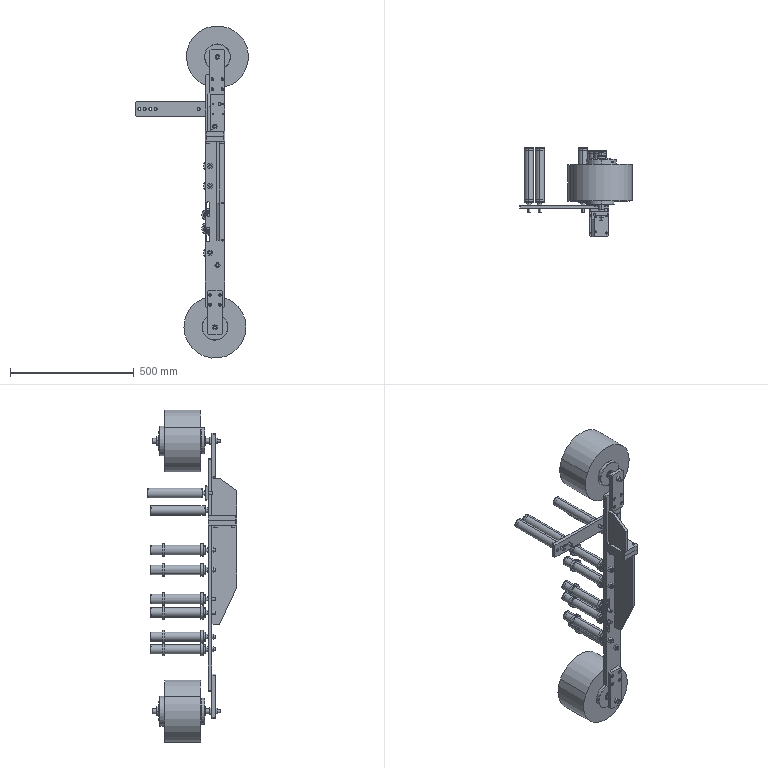Assembly | SolidWorks | mm | 137 component files | 139 solids | 2845 faces | box 455 x 361 x 1340 mm | volume 19278067 mm3 | cylinder 1536 | plane 969 | cone 300 | torus 40 | commonest cylinder face diameters 32 x120 15 x104 33.7 x100 6 x96 28 x80 19 x80 2.5 x80 12 x70
Bill of materials:
8TC-A15004-40-23A | 2 | A3 | Thick annular ring (short hollow cylinder) with small chamfers on its outer edges and one small radial hole through the wall.
8TC-A15004-40-25A | 2 | A3 | Thin flat annular disc (washer-like) with a large central through hole and square-cut edges.
8TC-A15004-80-01A | 1 | A3 | Long, narrow, thin rectangular bar with many through holes of several sizes, two elongated slots, and two blind holes drilled into one narrow end face.
8TC-A15004-80-02A | 2 | A3 | Thick rectangular block plate with two chamfered corners at one end and eight vertical through holes in two sizes.
8TC-A15004-80-03A | 1 | A3 | Flat rectangular bar with one end cut at an angle into a tapered tip, plus two blind holes drilled into the opposite narrow end face.
8TC-A15004-80-04A | 1 | A3 | Flat plate with a five-sided (pentagonal) outline formed by one large angled corner cut. No holes are visible.
8TC-A15004-80-05A | 1 | A3 | Rectangular plate with two chamfered corners at one end and about 13 through holes in roughly three sizes, laid out in a pattern.
8TC-A15004-80-15A | 2 | A3 | Rectangular plate with all four corners chamfered, one larger through hole near one end, and four smaller through holes in a rectangular pattern near the other end.
8TC-A15004-80-16A | 2 | #45 | Stepped cylindrical pin: a long main shaft, a short larger-diameter collar, and a short smaller-diameter stub at one end. The collar appears to have two parallel flats.
8TC-A15004-80-17A | 2 | Black POM | Flanged cylindrical sleeve: a plain cylinder with a thin, larger-diameter flange at one end and a small axial through hole.
8TC-A15004-80-18A | 2 | Black POM | Split ring: an annulus with a single radial slit through the wall and a transverse hole crossing the split region perpendicular to the slit.
8TC-A15004-80-19A | 12 | Black Bakelite | Thin-walled annular ring with small edge chamfers and small radial hole(s) through the wall.
6002 | 20 |  | Short annular ring: a cylinder with a large central through bore and a thin concentric circular line on the end face between the bore and the outer edge.
8TC-A15004-80-13A | 10 | #45 | Long, straight, thin-walled cylindrical tube that is open along its full length.
8TC-A15004-80-14A | 10 | #45 | Long, slender, stepped round shaft. One end has a short small-diameter pin, then a short larger-diameter collar, then a long main shaft that ends in a short reduced or chamfered section.
circlips for hole--type b gb | 20 |  | Thin, flat, open split ring (C-shape) with a circular outer edge and a gap on one side. At each end of the gap the band widens inward into a lug with a small round through-hole. Shape resembles an internal-style retaining ring.
circlips for shaft--type a large gb | 10 |  | Thin, flat, open split ring (C-shape) with a circular inner edge and a narrow straight-sided gap on one side. At each end of the gap the band widens outward into a lug with a small round through-hole. Shape resembles an external-style retaining ring.
M12Nut | 7 | #45 | Hexagonal prism with a plain round through bore on its central axis.
M6x20SocketHeadCapScrew | 23 | #45 | Headed cylindrical pin: a short, larger-diameter cylindrical head joined to a longer, smaller-diameter cylindrical shank with a chamfered free end.
M8x30HexSocketHeadCapScrew | 4 | #45 | Headed cylindrical pin, similar to the previous part: a cylindrical head and a longer, smaller cylindrical shank with a chamfered end. The head is slightly smaller relative to the shank.
Part41 | 1 |  | Flat rectangular bar with small corner chamfers. It has a row of four round through holes near one end, one isolated round hole further along, and four lengthwise slots arranged in a 2x2 pattern near the other end.
ProtectiveFilm | 1 |  | Thick-walled cylindrical bushing or spacer shape: a solid cylinder with a small central through bore.
Mates:
1. coincident | 8TC-A15004-80-01A-1 face at (80, 7.5, 0) dir (0, 0, 1) | 8TC-A15004-80-02A-1 face at (40, -50, 0) dir (0, 0, -1)
2. width | 8TC-A15004-80-01A-1 face at (80, 7.5, -670) dir (1, 0, 0) | 8TC-A15004-80-01A-1 face at (0, 7.5, 0) dir (-1, 0, 0) | 8TC-A15004-80-02A-1 face at (80, -107.5, 0) dir (1, 0, 0) | 8TC-A15004-80-02A-1 face at (0, -107.5, 0) dir (-1, 0, 0)
3. coincident | 8TC-A15004-80-02A-1 face at (40, -50, 0) dir (0, 0, -1) | 8TC-A15004-80-03A-1 face at (60, -107.5, 0) dir (0, 0, 1)
4. coincident | 8TC-A15004-80-01A-1 face at (0, -7.5, 0) dir (0, -1, 0) | 8TC-A15004-80-03A-1 face at (60, -7.5, 0) dir (0, 1, 0)
5. coincident | 8TC-A15004-80-02A-1 face at (0, 7.5, 0) dir (0, 1, 0) | 8TC-A15004-80-02A-2 face at (80, 7.5, 40) dir (0, 1, 0)
6. coincident | 8TC-A15004-80-02A-2 face at (40, -50, 40) dir (0, 0, 1) | 8TC-A15004-80-05A-1 face at (80, -7.5, 40) dir (0, 0, -1)
7. coincident | 8TC-A15004-80-02A-2 face at (80, 7.5, 40) dir (0, 1, 0) | 8TC-A15004-80-05A-1 face at (0, 7.5, 40) dir (0, 1, 0)
8. coincident | 8TC-A15004-80-02A-2 face at (0, -107.5, 40) dir (-1, 0, 0) | 8TC-A15004-80-05A-1 face at (0, -7.5, 40) dir (-1, 0, 0)
9. distance | ProtectiveFilm-1 face at (40, 37.5, -750) dir (0, -1, 0) | 8TC-A15004-80-01A-1 face at (0, 7.5, 0) dir (0, 1, 0)
10. coincident | ProtectiveFilm-1 face at (40, 183.5, -750) dir (0, 1, 0) | ProtectiveFilm-4 face at (50, 183.5, 340) dir (0, 1, 0)
11. concentric | 8TC-A15004-80-01A-1 face at (50, -7.5, -500) dir (0, 1, 0) r 6 | 8TC-A15004-83-00-8/8TC-A15004-80-14A-1 face at (50, -22.5, -500) dir (0, -1, 0) r 6
12. coincident | 8TC-A15004-80-01A-1 face at (0, 7.5, 0) dir (0, 1, 0) | 8TC-A15004-83-00-8/8TC-A15004-80-14A-1 face at (50, 7.5, -505) dir (0, -1, 0)
13. concentric | 8TC-A15004-80-01A-1 face at (20, -7.5, -450) dir (0, 1, 0) r 6 | 8TC-A15004-83-00-9/8TC-A15004-80-14A-1 face at (20, -22.5, -450) dir (0, -1, 0) r 6
14. coincident | 8TC-A15004-80-01A-1 face at (0, 7.5, 0) dir (0, 1, 0) | 8TC-A15004-83-00-9/8TC-A15004-80-14A-1 face at (20, 7.5, -455) dir (0, -1, 0)
15. coincident | 8TC-A15004-80-05A-1 face at (0, 7.5, 40) dir (0, 1, 0) | assembly face at (20, 7.5, 185) dir (0, -1, 0)
16. concentric | 8TC-A15004-80-05A-1 face at (20, 7.5, 190) dir (0, -1, 0) r 10 | assembly face at (20, -22.5, 190) dir (0, -1, 0) r 6
17. coincident | 8TC-A15004-80-01A-1 face at (0, 7.5, 0) dir (0, 1, 0) | assembly face at (40, 7.5, -101.842) dir (0, -1, 0)
18. width | 8TC-A15004-80-01A-1 face at (0, 7.5, 0) dir (-1, 0, 0) | 8TC-A15004-80-01A-1 face at (80, 7.5, -670) dir (1, 0, 0) | assembly face at (15, 22.5, -26.842) dir (-1, 0, 0) | assembly face at (65, 22.5, -26.842) dir (1, 0, 0)
19. coincident | 8TC-A15004-80-01A-1 face at (0, 7.5, 0) dir (0, 1, 0) | assembly face at (40, 7.5, -325) dir (0, -1, 0)
20. width | 8TC-A15004-80-01A-1 face at (80, 7.5, -670) dir (1, 0, 0) | 8TC-A15004-80-01A-1 face at (0, 7.5, 0) dir (-1, 0, 0) | assembly face at (0, 22.5, -415) dir (-1, 0, 0) | assembly face at (80, 22.5, -415) dir (1, 0, 0)
21. distance | assembly face at (80, 22.5, -235) dir (0, 0, 1) | 8TC-A15004-80-02A-1 face at (40, -50, 20) dir (0, 0, 1)
22. concentric | 8TC-A15004-80-01A-1 face at (20, -7.5, -100) dir (0, 1, 0) r 6 | 8TC-A15004-83-00-7/8TC-A15004-80-14A-1 face at (20, -22.5, -100) dir (0, -1, 0) r 6
23. concentric | 8TC-A15004-80-01A-1 face at (20, -7.5, -180) dir (0, 1, 0) r 6 | 8TC-A15004-83-00-6/8TC-A15004-80-14A-1 face at (20, -22.5, -180) dir (0, -1, 0) r 6
24. coincident | 8TC-A15004-80-01A-1 face at (0, 7.5, 0) dir (0, 1, 0) | 8TC-A15004-83-00-6/8TC-A15004-80-14A-1 face at (20, 7.5, -185) dir (0, -1, 0)
25. coincident | 8TC-A15004-80-01A-1 face at (0, 7.5, 0) dir (0, 1, 0) | 8TC-A15004-83-00-7/8TC-A15004-80-14A-1 face at (20, 7.5, -105) dir (0, -1, 0)
26. distance | 8TC-A15004-80-03A-1 face at (60, -7.5, 0) dir (1, 0, 0) | 8TC-A15004-80-01A-1 face at (80, 7.5, -670) dir (1, 0, 0)
27. coincident | 8TC-A15004-80-05A-1 face at (0, -7.5, 40) dir (0, -1, 0) | 8TC-A15004-80-04A-1 face at (10, -7.5, 40) dir (0, 1, 0)
28. coincident | 8TC-A15004-80-02A-2 face at (40, -50, 40) dir (0, 0, 1) | 8TC-A15004-80-04A-1 face at (10, -107.5, 40) dir (0, 0, -1)
29. distance | 8TC-A15004-80-04A-1 face at (10, -7.5, 40) dir (-1, 0, 0) | 8TC-A15004-80-02A-2 face at (0, -107.5, 40) dir (-1, 0, 0)
30. concentric | 8TC-A15004-80-02A-2 face at (26, -87.5, 20) dir (0, 0, -1) r 3.3 | M6x20SocketHeadCapScrew-1 face at (26, -87.5, 46.4) dir (0, 0, 1) r 3
31. coincident | 8TC-A15004-80-02A-2 face at (26, -84.2, 26.4) dir (0, 0, -1) | M6x20SocketHeadCapScrew-1 face at (20.75, -87.5, 26.4) dir (0, 0, 1)
32. concentric | 8TC-A15004-80-02A-2 face at (26, -27.5, 20) dir (0, 0, -1) r 3.3 | M6x20SocketHeadCapScrew-2 face at (26, -27.5, 46.4) dir (0, 0, 1) r 3
33. coincident | 8TC-A15004-80-02A-2 face at (26, -24.2, 26.4) dir (0, 0, -1) | M6x20SocketHeadCapScrew-2 face at (20.75, -27.5, 26.4) dir (0, 0, 1)
34. concentric | 8TC-A15004-80-02A-2 face at (20, 0, 20) dir (0, 0, -1) r 3.3 | M6x20SocketHeadCapScrew-3 face at (20, 0, 46.4) dir (0, 0, 1) r 3
35. coincident | M6x20SocketHeadCapScrew-2 face at (26, -27.5, 20.4) dir (0, 0, -1) | M6x20SocketHeadCapScrew-3 face at (20, 0, 20.4) dir (0, 0, -1)
36. concentric | 8TC-A15004-80-02A-2 face at (60, 0, 20) dir (0, 0, -1) r 3.3 | M6x20SocketHeadCapScrew-4 face at (60, 0, 46.4) dir (0, 0, 1) r 3
37. coincident | M6x20SocketHeadCapScrew-3 face at (20, 0, 20.4) dir (0, 0, -1) | M6x20SocketHeadCapScrew-4 face at (60, 0, 20.4) dir (0, 0, -1)
38. coincident | 8TC-A15004-80-05A-1 face at (19.3, 1.1, 70) dir (0, 1, 0) | M6x20SocketHeadCapScrew-5 face at (10.75, 1.1, 70) dir (0, -1, 0)
39. concentric | 8TC-A15004-80-05A-1 face at (16, 7.5, 70) dir (0, 1, 0) r 3.3 | M6x20SocketHeadCapScrew-5 face at (16, -18.9, 70) dir (0, -1, 0) r 3
40. coincident | M6x20SocketHeadCapScrew-5 face at (16, 7.1, 70) dir (0, 1, 0) | M6x20SocketHeadCapScrew-6 face at (16, 7.1, 120) dir (0, 1, 0)
41. concentric | 8TC-A15004-80-05A-1 face at (16, 7.5, 120) dir (0, 1, 0) r 3.3 | M6x20SocketHeadCapScrew-6 face at (16, -18.9, 120) dir (0, -1, 0) r 3
42. coincident | M6x20SocketHeadCapScrew-6 face at (16, 7.1, 120) dir (0, 1, 0) | M6x20SocketHeadCapScrew-7 face at (16, 7.1, 170) dir (0, 1, 0)
43. concentric | 8TC-A15004-80-05A-1 face at (16, 7.5, 170) dir (0, 1, 0) r 3.3 | M6x20SocketHeadCapScrew-7 face at (16, -18.9, 170) dir (0, -1, 0) r 3
44. coincident | 8TC-A15004-80-05A-1 face at (0, -7.5, 40) dir (0, -1, 0) | M12Nut-1 face at (40, -7.5, 60) dir (0, 1, 0)
45. coincident | 8TC-A15004-80-01A-1 face at (0, -7.5, 0) dir (0, -1, 0) | M12Nut-2 face at (20, -7.5, -100) dir (0, 1, 0)
46. concentric | 8TC-A15004-83-00-7/8TC-A15004-80-14A-1 face at (20, -22.5, -100) dir (0, -1, 0) r 6 | M12Nut-2 face at (20, -7.5, -100) dir (0, 1, 0) r 6
47. coincident | 8TC-A15004-80-01A-1 face at (0, -7.5, 0) dir (0, -1, 0) | M12Nut-13 face at (20, -7.5, -180) dir (0, 1, 0)
48. concentric | 8TC-A15004-83-00-6/8TC-A15004-80-14A-1 face at (20, -22.5, -180) dir (0, -1, 0) r 6 | M12Nut-13 face at (20, -7.5, -180) dir (0, 1, 0) r 6
49. concentric | 8TC-A15004-83-00-9/8TC-A15004-80-14A-1 face at (20, -22.5, -450) dir (0, -1, 0) r 6 | M12Nut-15 face at (20, -7.5, -450) dir (0, 1, 0) r 6
50. coincident | 8TC-A15004-80-01A-1 face at (0, -7.5, 0) dir (0, -1, 0) | M12Nut-15 face at (20, -7.5, -450) dir (0, 1, 0)
51. coincident | 8TC-A15004-80-01A-1 face at (0, -7.5, 0) dir (0, -1, 0) | M12Nut-17 face at (50, -7.5, -500) dir (0, 1, 0)
52. concentric | 8TC-A15004-83-00-8/8TC-A15004-80-14A-1 face at (50, -22.5, -500) dir (0, -1, 0) r 6 | M12Nut-17 face at (50, -7.5, -500) dir (0, 1, 0) r 6
53. coincident | 8TC-A15004-80-02A-1 face at (40, -50, 0) dir (0, 0, -1) | M8x30HexSocketHeadCapScrew-5 face at (3, -92.5, 0) dir (0, 0, 1)
54. concentric | 8TC-A15004-80-02A-1 face at (10, -92.5, 0) dir (0, 0, -1) r 4.5 | M8x30HexSocketHeadCapScrew-5 face at (10, -92.5, 30) dir (0, 0, 1) r 4
55. coincident | 8TC-A15004-80-02A-1 face at (40, -50, 0) dir (0, 0, -1) | M8x30HexSocketHeadCapScrew-13 face at (63, -92.5, 0) dir (0, 0, 1)
56. concentric | 8TC-A15004-80-02A-1 face at (70, -92.5, 0) dir (0, 0, -1) r 4.5 | M8x30HexSocketHeadCapScrew-13 face at (70, -92.5, 30) dir (0, 0, 1) r 4
57. coincident | 8TC-A15004-80-02A-1 face at (40, -50, 0) dir (0, 0, -1) | M8x30HexSocketHeadCapScrew-15 face at (3, -22.5, 0) dir (0, 0, 1)
58. concentric | 8TC-A15004-80-02A-1 face at (10, -22.5, 0) dir (0, 0, -1) r 4.5 | M8x30HexSocketHeadCapScrew-15 face at (10, -22.5, 30) dir (0, 0, 1) r 4
59. concentric | 8TC-A15004-80-02A-1 face at (70, -22.5, 0) dir (0, 0, -1) r 4.5 | M8x30HexSocketHeadCapScrew-17 face at (70, -22.5, 30) dir (0, 0, 1) r 4
60. coincident | 8TC-A15004-80-02A-1 face at (40, -50, 0) dir (0, 0, -1) | M8x30HexSocketHeadCapScrew-17 face at (63, -22.5, 0) dir (0, 0, 1)
61. coincident | 8TC-A15004-80-02A-1 face at (54, -84.2, 13.6) dir (0, 0, 1) | M6x20SocketHeadCapScrew-8 face at (58.85, -85.489, 13.6) dir (0, 0, -1)
62. concentric | 8TC-A15004-80-02A-1 face at (54, -87.5, 20) dir (0, 0, 1) r 3.3 | M6x20SocketHeadCapScrew-8 face at (54, -87.5, -6.4) dir (0, 0, -1) r 3
63. coincident | M6x20SocketHeadCapScrew-8 face at (54, -87.5, 19.6) dir (0, 0, 1) | M6x20SocketHeadCapScrew-40 face at (54, -27.5, 19.6) dir (0, 0, 1)
64. concentric | 8TC-A15004-80-02A-1 face at (54, -27.5, 20) dir (0, 0, 1) r 3.3 | M6x20SocketHeadCapScrew-40 face at (54, -27.5, -6.4) dir (0, 0, -1) r 3
65. coincident | M6x20SocketHeadCapScrew-40 face at (54, -27.5, 19.6) dir (0, 0, 1) | M6x20SocketHeadCapScrew-42 face at (60, 0, 19.6) dir (0, 0, 1)
66. concentric | 8TC-A15004-80-02A-1 face at (60, 0, 20) dir (0, 0, 1) r 3.3 | M6x20SocketHeadCapScrew-42 face at (60, 0, -6.4) dir (0, 0, -1) r 3
67. coincident | M6x20SocketHeadCapScrew-42 face at (60, 0, 19.6) dir (0, 0, 1) | M6x20SocketHeadCapScrew-44 face at (20, 0, 19.6) dir (0, 0, 1)
68. concentric | 8TC-A15004-80-02A-1 face at (20, 0, 20) dir (0, 0, 1) r 3.3 | M6x20SocketHeadCapScrew-44 face at (20, 0, -6.4) dir (0, 0, -1) r 3
69. coincident | 8TC-A15004-80-01A-1 face at (57.3, 1.1, -50) dir (0, 1, 0) | M6x20SocketHeadCapScrew-46 face at (59.09, 1.1, -51.288) dir (0, -1, 0)
70. concentric | 8TC-A15004-80-01A-1 face at (54, 7.5, -50) dir (0, 1, 0) r 3.3 | M6x20SocketHeadCapScrew-46 face at (54, -18.9, -50) dir (0, -1, 0) r 3
71. coincident | M6x20SocketHeadCapScrew-46 face at (54, 7.1, -50) dir (0, 1, 0) | M6x20SocketHeadCapScrew-48 face at (54, 7.1, -150) dir (0, 1, 0)
72. concentric | 8TC-A15004-80-01A-1 face at (54, 7.5, -150) dir (0, 1, 0) r 3.3 | M6x20SocketHeadCapScrew-48 face at (54, -18.9, -150) dir (0, -1, 0) r 3
73. coincident | M6x20SocketHeadCapScrew-48 face at (54, 7.1, -150) dir (0, 1, 0) | M6x20SocketHeadCapScrew-50 face at (54, 7.1, -250) dir (0, 1, 0)
74. concentric | 8TC-A15004-80-01A-1 face at (54, 7.5, -250) dir (0, 1, 0) r 3.3 | M6x20SocketHeadCapScrew-50 face at (54, -18.9, -250) dir (0, -1, 0) r 3
75. coincident | M6x20SocketHeadCapScrew-50 face at (54, 7.1, -250) dir (0, 1, 0) | M6x20SocketHeadCapScrew-52 face at (54, 7.1, -350) dir (0, 1, 0)
76. concentric | 8TC-A15004-80-01A-1 face at (54, 7.5, -350) dir (0, 1, 0) r 3.3 | M6x20SocketHeadCapScrew-52 face at (54, -18.9, -350) dir (0, -1, 0) r 3
77. coincident | assembly face at (40, 236.5, -320) dir (0, 1, 0) | assembly face at (22.25, 236.5, -385) dir (0, -1, 0)
78. concentric | assembly face at (27.5, 236.5, -385) dir (0, 1, 0) r 3.3 | assembly face at (27.5, 216.5, -385) dir (0, -1, 0) r 3
79. concentric | assembly face at (52.5, 236.5, -385) dir (0, 1, 0) r 3.3 | assembly face at (52.5, 216.5, -385) dir (0, -1, 0) r 3
80. coincident | assembly face at (40, 236.5, -320) dir (0, 1, 0) | assembly face at (47.25, 236.5, -385) dir (0, -1, 0)
81. concentric | assembly face at (27.5, 236.5, -255) dir (0, 1, 0) r 3.3 | assembly face at (27.5, 216.5, -255) dir (0, -1, 0) r 3
82. coincident | assembly face at (40, 236.5, -320) dir (0, 1, 0) | assembly face at (22.25, 236.5, -255) dir (0, -1, 0)
83. coincident | assembly face at (40, 236.5, -320) dir (0, 1, 0) | assembly face at (47.25, 236.5, -255) dir (0, -1, 0)
84. concentric | assembly face at (52.5, 236.5, -255) dir (0, 1, 0) r 3.3 | assembly face at (52.5, 216.5, -255) dir (0, -1, 0) r 3
85. coincident | assembly face at (49.2, 31.1, -320) dir (0, 1, 0) | assembly face at (47.25, 31.1, -320) dir (0, -1, 0)
86. concentric | assembly face at (52.5, 37.5, -320) dir (0, 1, 0) r 3.3 | assembly face at (52.5, 11.1, -320) dir (0, -1, 0) r 3
87. coincident | assembly face at (52.5, 37.1, -320) dir (0, 1, 0) | assembly face at (87.633, 37.1, -298.125) dir (0, 1, 0)
88. coincident | assembly face at (52.5, 37.1, -320) dir (0, 1, 0) | assembly face at (27.5, 37.1, -320) dir (0, 1, 0)
89. coincident | assembly face at (52.5, 37.1, -320) dir (0, 1, 0) | assembly face at (52.5, 37.1, -220) dir (0, 1, 0)
90. coincident | assembly face at (52.5, 37.1, -320) dir (0, 1, 0) | assembly face at (27.5, 37.1, -220) dir (0, 1, 0)
91. concentric | assembly face at (27.5, 11.1, -320) dir (0, -1, 0) r 3 | assembly face at (27.5, 37.5, -320) dir (0, 1, 0) r 3.3
92. concentric | assembly face at (52.5, 11.1, -220) dir (0, -1, 0) r 3 | assembly face at (52.5, 37.5, -220) dir (0, 1, 0) r 3.3
93. concentric | assembly face at (27.5, 37.5, -220) dir (0, 1, 0) r 3.3 | assembly face at (27.5, 11.1, -220) dir (0, -1, 0) r 3
94. concentric | ProtectiveFilm-1 face at (40, 183.5, -750) dir (0, -1, 0) r 38.5 | assembly face at (150, -7.5, -640) dir (0, -1, 0) r 7.5
95. coincident | 8TC-A15004-80-15A-4 face at (30, -16.1, 213.3) dir (0, -1, 0) | M6x20SocketHeadCapScrew-54 face at (25.605, -16.1, 207.129) dir (0, 1, 0)
96. concentric | 8TC-A15004-80-15A-4 face at (30, -22.5, 210) dir (0, -1, 0) r 3.3 | M6x20SocketHeadCapScrew-54 face at (30, 3.9, 210) dir (0, 1, 0) r 3
97. coincident | M6x20SocketHeadCapScrew-54 face at (30, -22.1, 210) dir (0, -1, 0) | M6x20SocketHeadCapScrew-55 face at (70, -22.1, 250) dir (0, -1, 0)
98. coincident | M6x20SocketHeadCapScrew-55 face at (70, -22.1, 250) dir (0, -1, 0) | M6x20SocketHeadCapScrew-56 face at (70, -22.1, 210) dir (0, -1, 0)
99. coincident | M6x20SocketHeadCapScrew-55 face at (70, -22.1, 250) dir (0, -1, 0) | M6x20SocketHeadCapScrew-57 face at (30, -22.1, 250) dir (0, -1, 0)
100. concentric | 8TC-A15004-80-15A-4 face at (30, -22.5, 250) dir (0, -1, 0) r 3.3 | M6x20SocketHeadCapScrew-57 face at (30, 3.9, 250) dir (0, 1, 0) r 3
101. coincident | 8TC-A15004-80-15A-5 face at (20, -16.1, -623.3) dir (0, -1, 0) | M6x20SocketHeadCapScrew-58 face at (15.605, -16.1, -662.871) dir (0, 1, 0)
102. coincident | 8TC-A15004-80-15A-5 face at (60, -16.1, -623.3) dir (0, -1, 0) | M6x20SocketHeadCapScrew-60 face at (15.605, -16.1, -622.871) dir (0, 1, 0)
103. coincident | 8TC-A15004-80-15A-5 face at (60, -16.1, -663.3) dir (0, -1, 0) | M6x20SocketHeadCapScrew-62 face at (55.605, -16.1, -622.871) dir (0, 1, 0)
104. coincident | 8TC-A15004-80-15A-5 face at (20, -16.1, -663.3) dir (0, -1, 0) | M6x20SocketHeadCapScrew-64 face at (55.605, -16.1, -662.871) dir (0, 1, 0)
105. concentric | 8TC-A15004-80-15A-4 face at (50, -7.5, 340) dir (0, -1, 0) r 6 | 8TC-A15004-80-16A-4 face at (50, -42.5, 340) dir (0, -1, 0) r 6
106. coincident | 8TC-A15004-80-01A-1 face at (0, -7.5, 0) dir (0, -1, 0) | 8TC-A15004-80-15A-5 face at (40, -7.5, -690) dir (0, 1, 0)
107. coincident | 8TC-A15004-80-15A-5 face at (40, -22.5, -690) dir (0, -1, 0) | M12Nut-19 face at (40, -22.5, -750) dir (0, 1, 0)
108. concentric | 8TC-A15004-80-15A-5 face at (40, -7.5, -750) dir (0, -1, 0) r 6 | M12Nut-19 face at (40, -30.5, -750) dir (0, -1, 0) r 6
109. coincident | 8TC-A15004-80-15A-5 face at (40, -7.5, -690) dir (0, 1, 0) | 8TC-A15004-80-16A-3 face at (40.526, -7.5, -745.028) dir (0, -1, 0)
110. concentric | 8TC-A15004-80-16A-3 face at (40, -42.5, -750) dir (0, -1, 0) r 6 | M12Nut-19 face at (40, -30.5, -750) dir (0, -1, 0) r 6
111. coincident | ProtectiveFilm-1 face at (40, 37.5, -750) dir (0, -1, 0) | 8TC-A15004-80-17A-1 face at (40, 37.5, -788.5) dir (0, 1, 0)
112. concentric | ProtectiveFilm-1 face at (40, 183.5, -750) dir (0, -1, 0) r 38.5 | 8TC-A15004-80-17A-1 face at (40, 22.5, -750) dir (0, -1, 0) r 38.5
113. concentric | 8TC-A15004-80-17A-1 face at (40, 22.5, -750) dir (0, -1, 0) r 38.5 | 8TC-A15004-80-18A-1 face at (40, 203.5, -750) dir (0, -1, 0) r 38.5
114. coincident | ProtectiveFilm-1 face at (40, 183.5, -750) dir (0, 1, 0) | 8TC-A15004-80-18A-1 face at (40, 183.5, -750) dir (0, -1, 0)
115. concentric | 8TC-A15004-80-16A-3 face at (40, -42.5, -750) dir (0, -1, 0) r 10 | 8TC-A15004-40-23A-1 face at (40, 207.5, -750) dir (0, 1, 0) r 10
116. coincident | 8TC-A15004-80-17A-1 face at (40, 207.5, -760) dir (0, 1, 0) | 8TC-A15004-40-23A-1 face at (40, 207.5, -750) dir (0, -1, 0)
117. concentric | 8TC-A15004-80-16A-3 face at (40, -42.5, -750) dir (0, -1, 0) r 10 | 8TC-A15004-40-25A-1 face at (40, 22.5, -750) dir (0, -1, 0) r 10.25
118. coincident | 8TC-A15004-80-17A-1 face at (40, 22.5, -802.5) dir (0, -1, 0) | 8TC-A15004-40-25A-1 face at (40, 22.5, -750) dir (0, 1, 0)
119. coincident | 8TC-A15004-80-05A-1 face at (0, -7.5, 40) dir (0, -1, 0) | 8TC-A15004-80-15A-4 face at (50, -7.5, 280) dir (0, 1, 0)
120. coincident | 8TC-A15004-80-15A-4 face at (50, -22.5, 280) dir (0, -1, 0) | M12Nut-21 face at (50, -22.5, 340) dir (0, 1, 0)
121. concentric | 8TC-A15004-80-15A-4 face at (50, -7.5, 340) dir (0, -1, 0) r 6 | M12Nut-21 face at (50, -30.5, 340) dir (0, -1, 0) r 6
122. coincident | 8TC-A15004-80-15A-4 face at (50, -7.5, 280) dir (0, 1, 0) | 8TC-A15004-80-16A-4 face at (50, -7.5, 345) dir (0, -1, 0)
123. concentric | 8TC-A15004-80-16A-4 face at (50, -42.5, 340) dir (0, -1, 0) r 10 | 8TC-A15004-80-17A-2 face at (50, 22.5, 340) dir (0, -1, 0) r 38.5
124. coincident | ProtectiveFilm-4 face at (50, 37.5, 340) dir (0, -1, 0) | 8TC-A15004-80-17A-2 face at (50, 37.5, 301.5) dir (0, 1, 0)
125. concentric | 8TC-A15004-80-17A-2 face at (50, 22.5, 340) dir (0, -1, 0) r 38.5 | 8TC-A15004-80-18A-2 face at (50, 203.5, 340) dir (0, -1, 0) r 38.5
126. coincident | ProtectiveFilm-4 face at (50, 183.5, 340) dir (0, 1, 0) | 8TC-A15004-80-18A-2 face at (50, 183.5, 340) dir (0, -1, 0)
127. concentric | 8TC-A15004-80-16A-4 face at (50, -42.5, 340) dir (0, -1, 0) r 10 | 8TC-A15004-40-23A-2 face at (50, 207.5, 340) dir (0, 1, 0) r 10
128. coincident | 8TC-A15004-80-17A-2 face at (50, 207.5, 330) dir (0, 1, 0) | 8TC-A15004-40-23A-2 face at (50, 207.5, 340) dir (0, -1, 0)
129. coincident | 8TC-A15004-80-17A-2 face at (50, 22.5, 287.5) dir (0, -1, 0) | 8TC-A15004-40-25A-2 face at (50, 22.5, 340) dir (0, 1, 0)
130. concentric | 8TC-A15004-80-16A-4 face at (50, -42.5, 340) dir (0, -1, 0) r 10 | 8TC-A15004-40-25A-2 face at (50, 22.5, 340) dir (0, -1, 0) r 10.25
131. concentric | 8TC-A15004-83-00-8/8TC-A15004-80-13A-1 face at (50, 100.224, -500) dir (0, -1, 0) r 19 | 8TC-A15004-80-19A-1 face at (50, 193.5, -500) dir (0, -1, 0) r 19.05
132. coincident | ProtectiveFilm-1 face at (40, 183.5, -750) dir (0, 1, 0) | 8TC-A15004-80-19A-1 face at (50, 183.5, -500) dir (0, -1, 0)
133. concentric | 8TC-A15004-83-00-8/8TC-A15004-80-13A-1 face at (50, 100.224, -500) dir (0, -1, 0) r 19 | 8TC-A15004-80-19A-2 face at (50, 37.5, -500) dir (0, -1, 0) r 19.05
134. coincident | ProtectiveFilm-1 face at (40, 37.5, -750) dir (0, -1, 0) | 8TC-A15004-80-19A-2 face at (50, 37.5, -500) dir (0, 1, 0)
135. concentric | 8TC-A15004-83-00-9/8TC-A15004-80-13A-1 face at (20, 100.224, -450) dir (0, -1, 0) r 19 | 8TC-A15004-80-19A-3 face at (20, 193.5, -450) dir (0, -1, 0) r 19.05
136. coincident | 8TC-A15004-80-19A-1 face at (50, 183.5, -500) dir (0, -1, 0) | 8TC-A15004-80-19A-3 face at (20, 183.5, -450) dir (0, -1, 0)
137. concentric | 8TC-A15004-83-00-9/8TC-A15004-80-13A-1 face at (20, 100.224, -450) dir (0, -1, 0) r 19 | 8TC-A15004-80-19A-4 face at (20, 37.5, -450) dir (0, -1, 0) r 19.05
138. coincident | 8TC-A15004-80-19A-2 face at (50, 37.5, -500) dir (0, 1, 0) | 8TC-A15004-80-19A-4 face at (20, 37.5, -450) dir (0, 1, 0)
139. concentric | 8TC-A15004-83-00-6/8TC-A15004-80-13A-1 face at (20, 100.224, -180) dir (0, -1, 0) r 19 | 8TC-A15004-80-19A-5 face at (20, 193.5, -180) dir (0, -1, 0) r 19.05
140. coincident | 8TC-A15004-80-19A-3 face at (20, 183.5, -450) dir (0, -1, 0) | 8TC-A15004-80-19A-5 face at (20, 183.5, -180) dir (0, -1, 0)
141. concentric | 8TC-A15004-83-00-6/8TC-A15004-80-13A-1 face at (20, 100.224, -180) dir (0, -1, 0) r 19 | 8TC-A15004-80-19A-6 face at (20, 37.5, -180) dir (0, -1, 0) r 19.05
142. coincident | 8TC-A15004-80-19A-4 face at (20, 37.5, -450) dir (0, 1, 0) | 8TC-A15004-80-19A-6 face at (20, 37.5, -180) dir (0, 1, 0)
143. concentric | 8TC-A15004-83-00-7/8TC-A15004-80-13A-1 face at (20, 100.224, -100) dir (0, -1, 0) r 19 | 8TC-A15004-80-19A-7 face at (20, 193.5, -100) dir (0, -1, 0) r 19.05
144. coincident | 8TC-A15004-80-19A-5 face at (20, 183.5, -180) dir (0, -1, 0) | 8TC-A15004-80-19A-7 face at (20, 183.5, -100) dir (0, -1, 0)
145. concentric | 8TC-A15004-83-00-7/8TC-A15004-80-13A-1 face at (20, 100.224, -100) dir (0, -1, 0) r 19 | 8TC-A15004-80-19A-8 face at (20, 37.5, -100) dir (0, -1, 0) r 19.05
146. coincident | 8TC-A15004-80-19A-6 face at (20, 37.5, -180) dir (0, 1, 0) | 8TC-A15004-80-19A-8 face at (20, 37.5, -100) dir (0, 1, 0)
147. concentric | 8TC-A15004-80-05A-1 face at (40, 7.5, 60) dir (0, 1, 0) r 6 | 8TC-A15004-83-00-16/8TC-A15004-80-14A-1 face at (40, -22.5, 60) dir (0, -1, 0) r 6
148. coincident | 8TC-A15004-80-05A-1 face at (0, 7.5, 40) dir (0, 1, 0) | 8TC-A15004-83-00-16/8TC-A15004-80-14A-1 face at (40, 7.5, 55) dir (0, -1, 0)
149. concentric | 8TC-A15004-80-01A-1 face at (20, 7.5, -620) dir (0, 1, 0) r 3 | 8TC-A15004-80-15A-5 face at (20, -22.5, -620) dir (0, -1, 0) r 3.3
150. concentric | 8TC-A15004-80-01A-1 face at (60, 7.5, -660) dir (0, 1, 0) r 3 | 8TC-A15004-80-15A-5 face at (60, -22.5, -660) dir (0, -1, 0) r 3.3
151. concentric | 8TC-A15004-80-16A-3 face at (40, -42.5, -750) dir (0, -1, 0) r 10 | 8TC-A15004-80-17A-1 face at (40, 22.5, -750) dir (0, -1, 0) r 10
152. distance | assembly face at (-590, 112.5, 90) dir (1, 0, 0) | 8TC-A15004-80-02A-3 face at (-530, -107.5, 0) dir (-1, 0, 0)
153. concentric | ProtectiveFilm-4 face at (50, 183.5, 340) dir (0, -1, 0) r 38.5 | 8TC-A15004-80-17A-2 face at (50, 22.5, 340) dir (0, -1, 0) r 38.5
154. concentric | M12Nut-1 face at (40, -7.5, 60) dir (0, 1, 0) r 6 | 8TC-A15004-83-00-16/8TC-A15004-80-14A-1 face at (40, -22.5, 60) dir (0, -1, 0) r 6
155. concentric | 8TC-A15004-80-05A-1 face at (70, 7.5, 250) dir (0, 1, 0) r 3 | M6x20SocketHeadCapScrew-55 face at (70, 3.9, 250) dir (0, 1, 0) r 3
156. distance | 8TC-A15004-80-05A-1 face at (0, -7.5, 270) dir (0, 0, 1) | 8TC-A15004-80-15A-4 face at (80, -22.5, 190) dir (0, 0, -1)
157. coincident | 8TC-A15004-80-05A-1 face at (80, -7.5, 270) dir (1, 0, 0) | 8TC-A15004-80-15A-4 face at (80, -22.5, 190) dir (1, 0, 0)
158. coincident | 8TC-A15004-80-01A-1 face at (0, 7.5, 0) dir (0, 1, 0) | 8TC-A15004-83-00-17/8TC-A15004-80-14A-1 face at (13, 7.5, -302.5) dir (0, -1, 0)
159. slot | 8TC-A15004-83-00-17/8TC-A15004-80-14A-1 face at (13, -22.5, -297.5) dir (0, -1, 0) r 6 | 8TC-A15004-80-01A-1 face at (19, -7.5, -297.5) dir (-1, 0, 0)
160. coincident | 8TC-A15004-80-01A-1 face at (0, 7.5, 0) dir (0, 1, 0) | 8TC-A15004-83-00-18/8TC-A15004-80-14A-1 face at (13, 7.5, -357.5) dir (0, -1, 0)
161. slot | 8TC-A15004-83-00-18/8TC-A15004-80-14A-1 face at (13, -22.5, -352.5) dir (0, -1, 0) r 6 | 8TC-A15004-80-01A-1 face at (19, -7.5, -352.5) dir (-1, 0, 0)
162. concentric | 8TC-A15004-83-00-18/8TC-A15004-80-13A-1 face at (13, 100.224, -352.5) dir (0, -1, 0) r 19 | 8TC-A15004-80-19A-17 face at (13, 193.5, -352.5) dir (0, -1, 0) r 19.05
163. coincident | 8TC-A15004-80-19A-3 face at (20, 193.5, -450) dir (0, 1, 0) | 8TC-A15004-80-19A-17 face at (13, 193.5, -352.5) dir (0, 1, 0)
164. concentric | 8TC-A15004-83-00-17/8TC-A15004-80-13A-1 face at (13, 100.224, -297.5) dir (0, -1, 0) r 19 | 8TC-A15004-80-19A-18 face at (13, 193.5, -297.5) dir (0, -1, 0) r 19.05
165. coincident | 8TC-A15004-80-19A-17 face at (13, 193.5, -352.5) dir (0, 1, 0) | 8TC-A15004-80-19A-18 face at (13, 193.5, -297.5) dir (0, 1, 0)
166. concentric | 8TC-A15004-83-00-17/8TC-A15004-80-13A-1 face at (13, 100.224, -297.5) dir (0, -1, 0) r 19 | 8TC-A15004-80-19A-19 face at (13, 37.5, -297.5) dir (0, -1, 0) r 19.05
167. coincident | 8TC-A15004-80-19A-4 face at (20, 27.5, -450) dir (0, -1, 0) | 8TC-A15004-80-19A-19 face at (13, 27.5, -297.5) dir (0, -1, 0)
168. concentric | 8TC-A15004-83-00-18/8TC-A15004-80-13A-1 face at (13, 100.224, -352.5) dir (0, -1, 0) r 19 | 8TC-A15004-80-19A-20 face at (13, 37.5, -352.5) dir (0, -1, 0) r 26
169. coincident | 8TC-A15004-80-19A-4 face at (20, 27.5, -450) dir (0, -1, 0) | 8TC-A15004-80-19A-20 face at (13, 27.5, -352.5) dir (0, -1, 0)
170. coincident | 8TC-A15004-80-05A-1 face at (0, 7.5, 40) dir (0, 1, 0) | Part41-1 face at (-100, 7.5, 130) dir (0, -1, 0)
171. coincident | 8TC-A15004-80-05A-1 face at (80, -7.5, 270) dir (1, 0, 0) | Part41-1 face at (80, 19.5, 160) dir (1, 0, 0)
172. distance | 8TC-A15004-80-02A-2 face at (40, -50, 20) dir (0, 0, -1) | Part41-1 face at (-280, 19.5, 100) dir (0, 0, -1)
173. concentric | Part41-1 face at (-25, -33.5, 130) dir (0, 1, 0) r 6 | 8TC-A15004-83-00-19/8TC-A15004-80-14A-1 face at (-25, -10.5, 130) dir (0, -1, 0) r 10
174. coincident | Part41-1 face at (-100, 19.5, 130) dir (0, 1, 0) | 8TC-A15004-83-00-19/8TC-A15004-80-14A-1 face at (-25, 19.5, 125) dir (0, -1, 0)
175. concentric | Part41-1 face at (-199, -33.5, 130) dir (0, 1, 0) r 6 | 8TC-A15004-83-00-20/8TC-A15004-80-14A-1 face at (-199, -10.5, 130) dir (0, -1, 0) r 10
176. coincident | Part41-1 face at (-100, 19.5, 130) dir (0, 1, 0) | 8TC-A15004-83-00-20/8TC-A15004-80-14A-1 face at (-199, 19.5, 125) dir (0, -1, 0)
177. concentric | Part41-1 face at (-243, -33.5, 130) dir (0, 1, 0) r 6 | 8TC-A15004-83-00-21/8TC-A15004-80-14A-1 face at (-243, -10.5, 130) dir (0, -1, 0) r 10
178. coincident | Part41-1 face at (-100, 19.5, 130) dir (0, 1, 0) | 8TC-A15004-83-00-21/8TC-A15004-80-14A-1 face at (-243, 19.5, 125) dir (0, -1, 0)
179. concentric | 8TC-A15004-80-02A-2 face at (10, -92.5, 40) dir (0, 0, 1) r 4.5 | M8x30HexSocketHeadCapScrew-5 face at (10, -92.5, 30) dir (0, 0, 1) r 4
180. concentric | 8TC-A15004-80-02A-1 face at (10, -92.5, 0) dir (0, 0, -1) r 4.5 | 8TC-A15004-80-02A-2 face at (10, -92.5, 40) dir (0, 0, 1) r 4.5
181. coincident | 8TC-A15004-80-02A-1 face at (40, -50, 20) dir (0, 0, 1) | 8TC-A15004-80-02A-2 face at (40, -50, 20) dir (0, 0, -1)
182. coincident | 8TC-A15004-80-02A-1 face at (0, -107.5, 0) dir (-1, 0, 0) | 8TC-A15004-80-02A-2 face at (0, -107.5, 40) dir (-1, 0, 0)
183. coincident | 8TC-A15004-80-02A-1 face at (40, -50, 20) dir (0, 0, 1) | 8TC-A15004-80-02A-2 face at (40, -50, 20) dir (0, 0, -1)
184. concentric | 8TC-A15004-80-15A-4 face at (70, -22.5, 210) dir (0, -1, 0) r 3.3 | M6x20SocketHeadCapScrew-56 face at (70, 3.9, 210) dir (0, 1, 0) r 3
185. coincident | 8TC-A15004-80-13A-1 face at (-78, 0, -15) dir (-1, 0, 0) | 6002-1 face at (-78, 0, 16) dir (1, 0, 0)
186. concentric | 8TC-A15004-80-13A-1 face at (-9.276, 0, 0) dir (-1, 0, 0) r 16 | 6002-1 face at (-82.5, 0, 0) dir (1, 0, 0) r 16
187. coincident | 8TC-A15004-80-13A-1 face at (119, 0, -15) dir (1, 0, 0) | 6002-2 face at (119, 0, -16) dir (-1, 0, 0)
188. concentric | 8TC-A15004-80-13A-1 face at (-9.276, 0, 0) dir (-1, 0, 0) r 16 | 6002-2 face at (123.5, 0, 0) dir (-1, 0, 0) r 16
189. coincident | 8TC-A15004-80-14A-1 face at (-87, 0, -10) dir (1, 0, 0) | 6002-1 face at (-87, 0, 9.5) dir (-1, 0, 0)
190. concentric | 8TC-A15004-80-14A-1 face at (-132, 0, 0) dir (-1, 0, 0) r 7.5 | 6002-1 face at (-82.5, 0, 0) dir (1, 0, 0) r 7.5
191. coincident | 8TC-A15004-80-14A-1 face at (128, 0, -7.5) dir (1, 0, 0) | circlips for shaft--type a large gb-1 face at (128, 0, 0) dir (-1, 0, 0)
192. concentric | 8TC-A15004-80-14A-1 face at (-132, 0, 0) dir (-1, 0, 0) r 6.9 | circlips for shaft--type a large gb-1 face at (129, 0, 0) dir (-1, 0, 0) r 6.9
193. coincident | 8TC-A15004-80-13A-1 face at (128, 0, -16) dir (1, 0, 0) | circlips for hole--type b gb-1 face at (128, 0, 0) dir (-1, 0, 0)
194. concentric | 8TC-A15004-80-13A-1 face at (-9.276, 0, 0) dir (-1, 0, 0) r 16.85 | circlips for hole--type b gb-1 face at (129.2, 0, 0) dir (-1, 0, 0) r 16.85
195. coincident | 8TC-A15004-80-13A-1 face at (-87, 0, -16) dir (-1, 0, 0) | circlips for hole--type b gb-2 face at (-87, 0, 0) dir (1, 0, 0)
196. concentric | 8TC-A15004-80-13A-1 face at (-9.276, 0, 0) dir (-1, 0, 0) r 16.85 | circlips for hole--type b gb-2 face at (-87, 0, 0) dir (-1, 0, 0) r 16.85